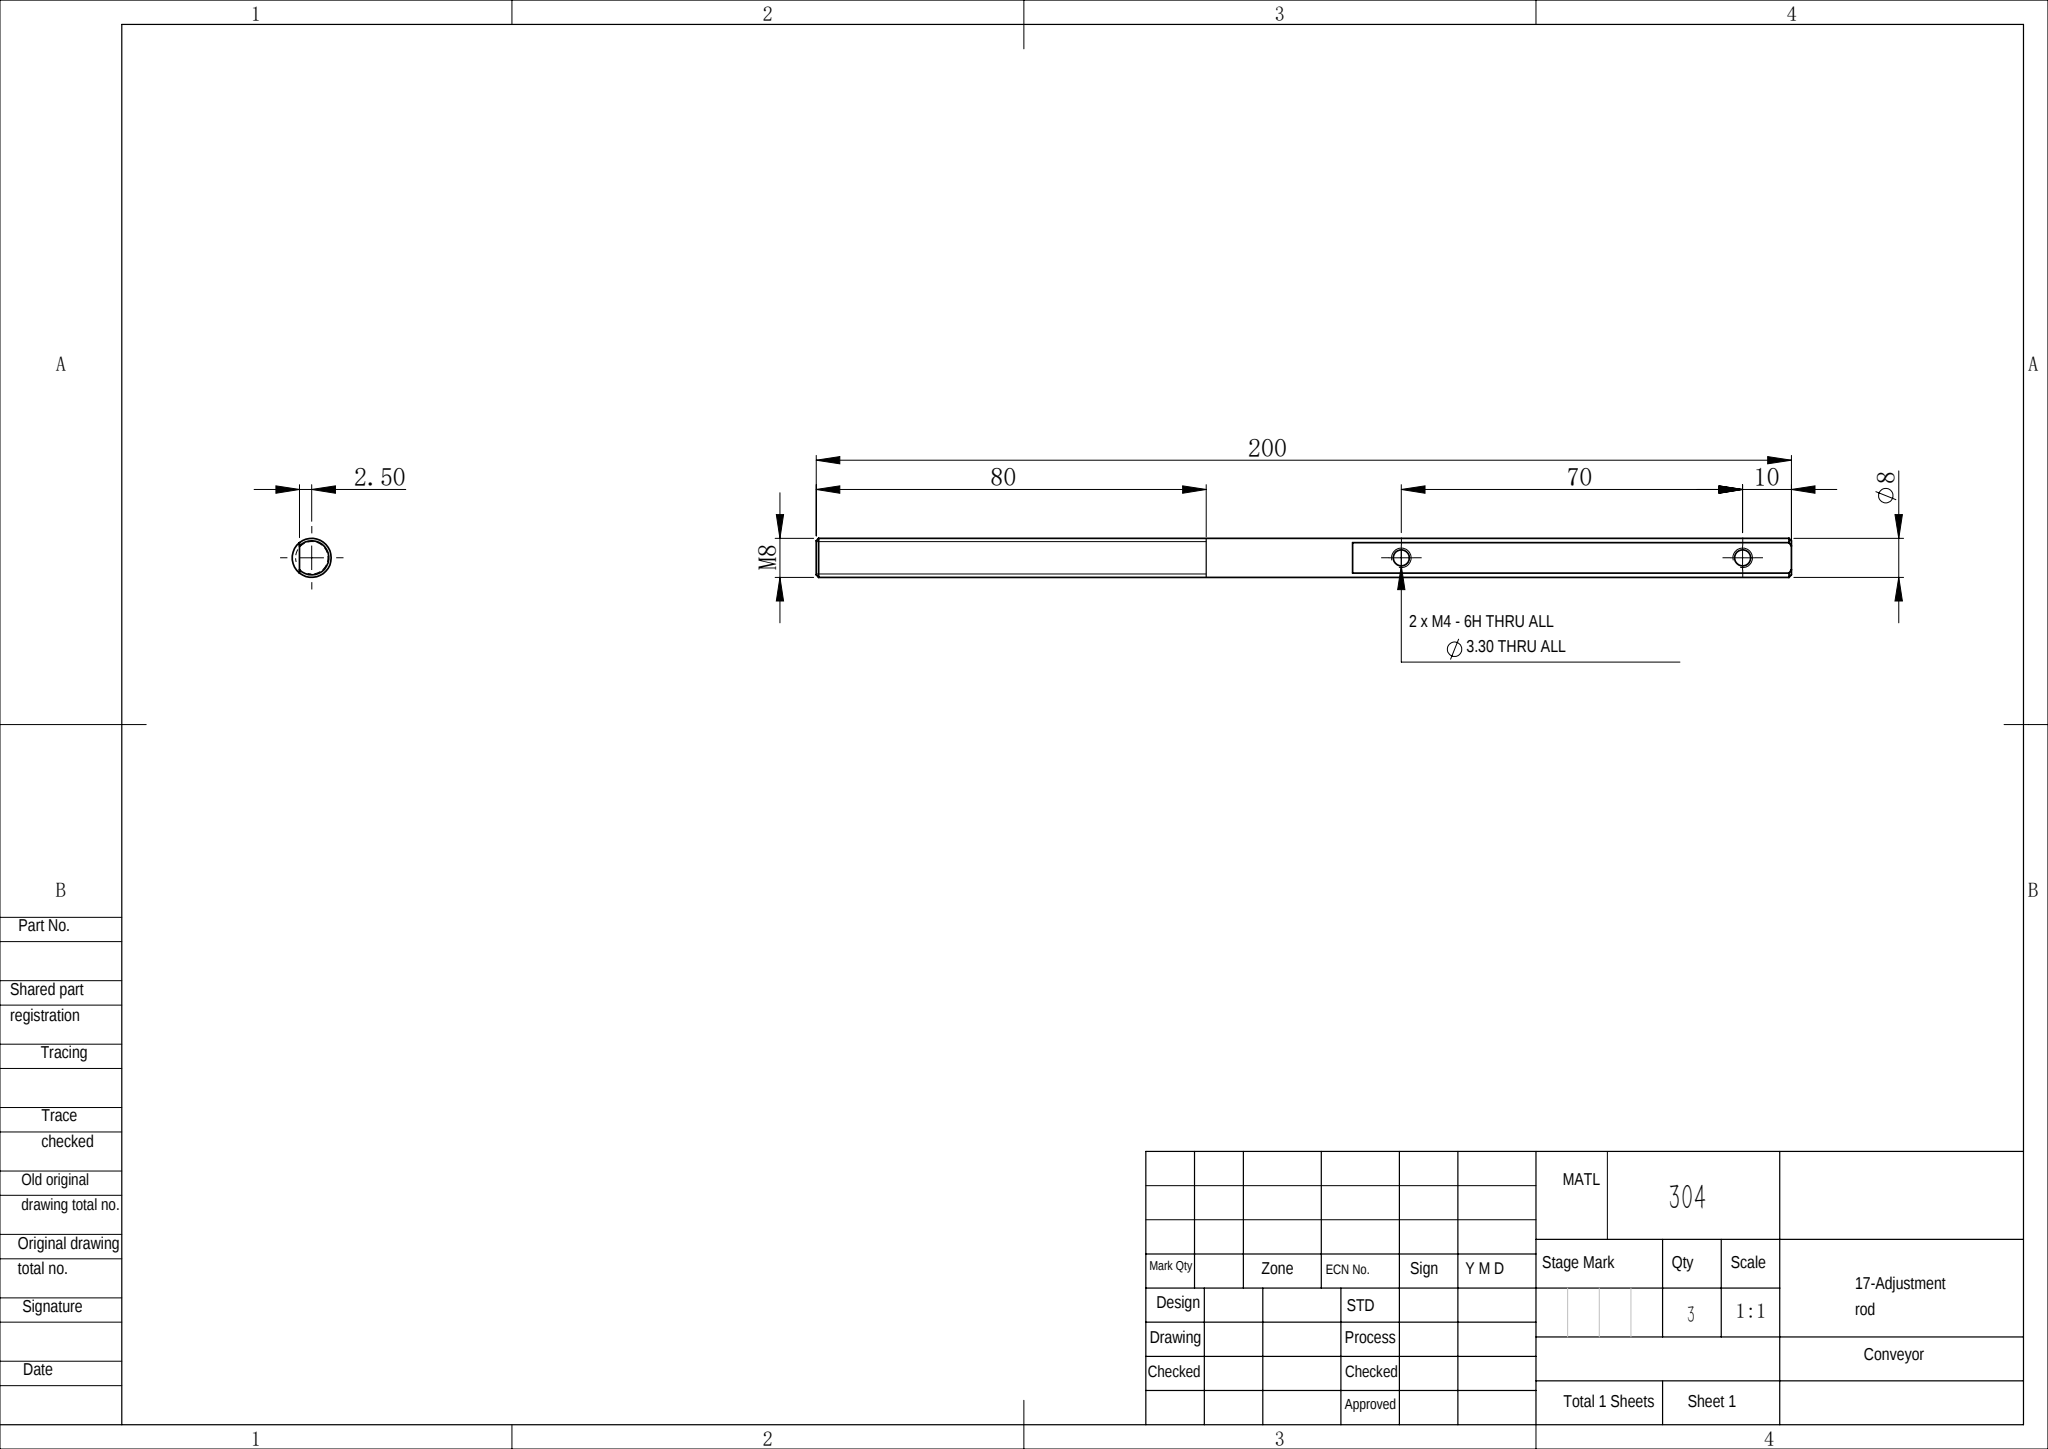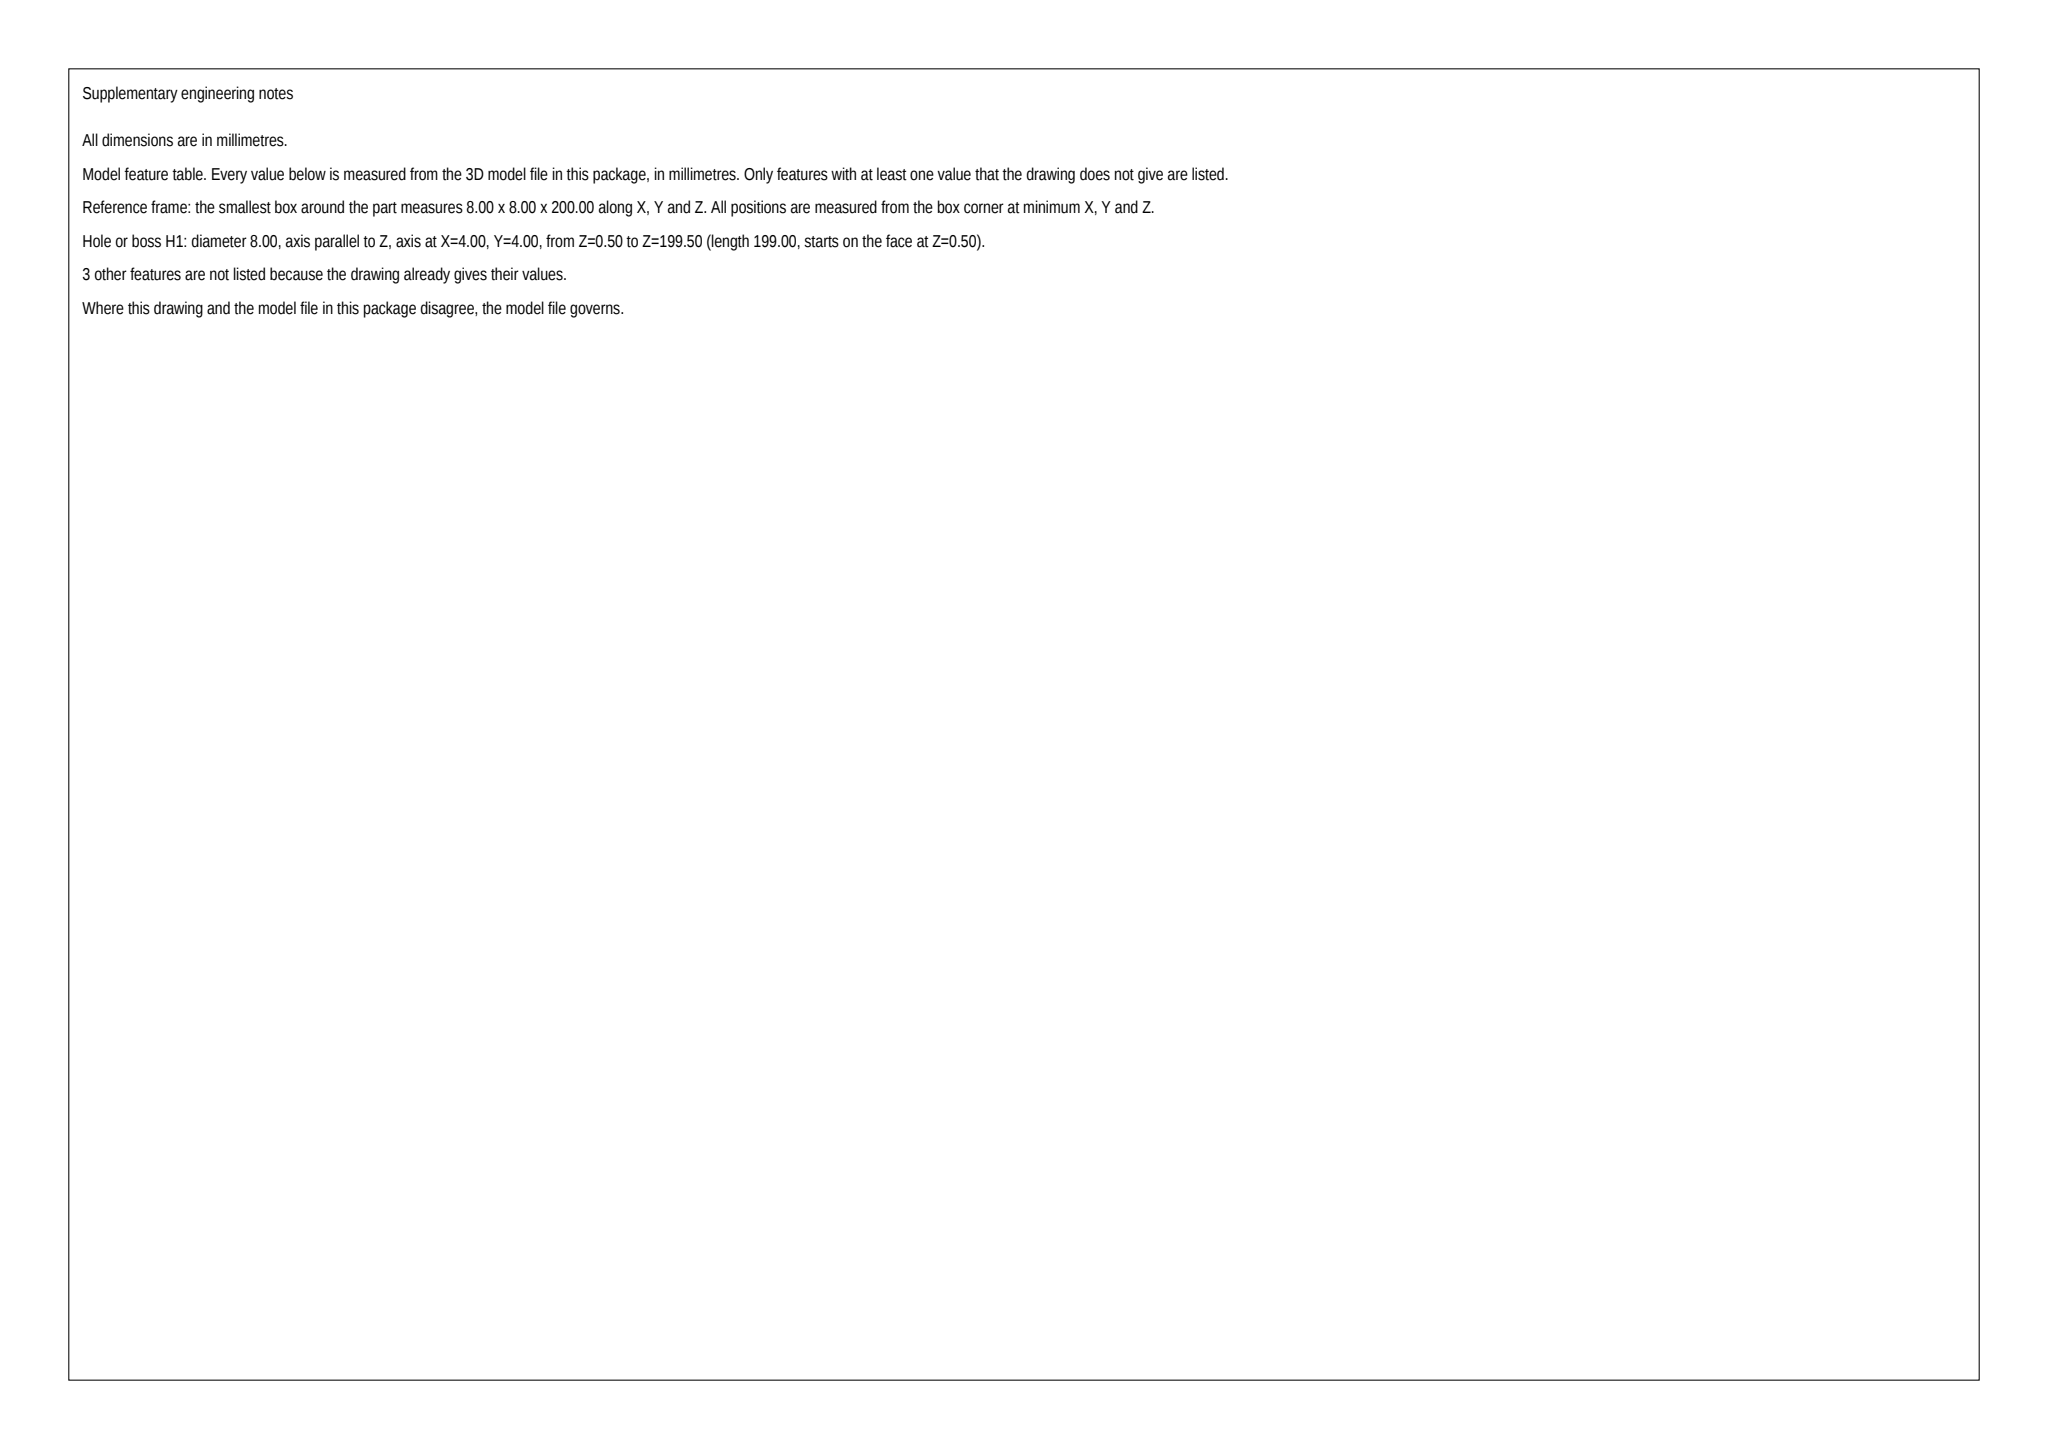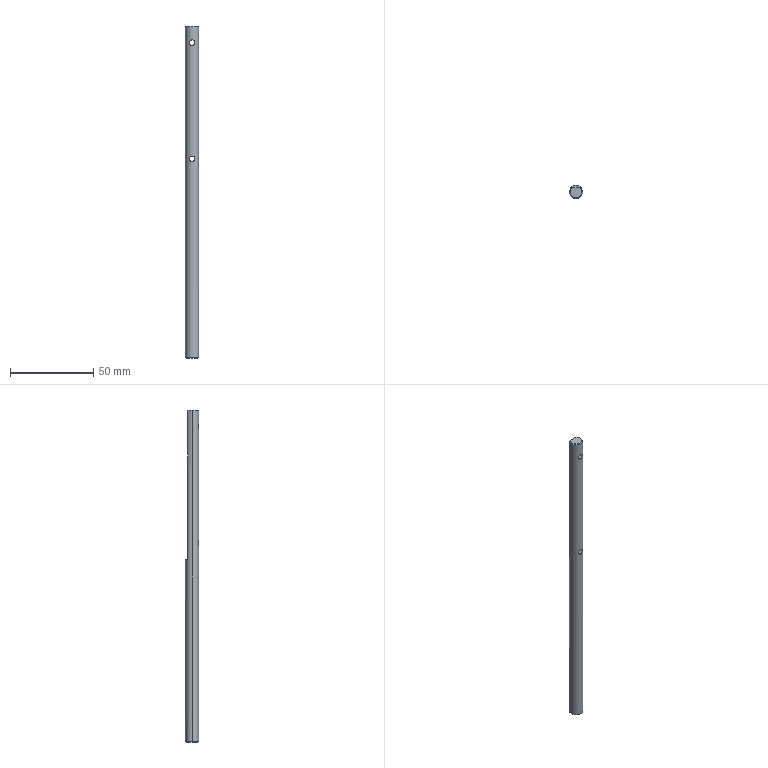Part | SolidWorks | mm | material 304 | 1 solid | 15 faces | box 8 x 8 x 200 mm | volume 9351 mm3 | cylinder 6 | cone 5 | plane 4 | commonest cylinder face diameters 3.3 x4 8 x2
build123d program:
from build123d import *

# Parameters (mm, degrees)
SKETCH1_R           = 4
BOSS_EXTRUDE1_DEPTH = 200
CHAMFER1_SIZE       = 0.5
SKETCH2_W           = 23.584
SKETCH2_H           = 6.641
CUT_EXTRUDE1_DEPTH  = 90
M4_TAPPED_HOLE1_D   = 3.3


with BuildPart() as part:
    # Sketch1 → Boss-Extrude1 (new body)
    with BuildSketch(Plane.XY):
        Circle(SKETCH1_R)
    extrude(amount=BOSS_EXTRUDE1_DEPTH)

    # Chamfer1
    chamfer1_edges = [part.edges().sort_by_distance(p)[0] for p in [
        (-4, 0, 0),
        (-4, 0, 200),
    ]]
    chamfer(chamfer1_edges, length=CHAMFER1_SIZE)

    # Sketch2 → Cut-Extrude1 (cut)
    with BuildSketch(Plane.XY.offset(200)):
        with Locations((0, 5.821)):
            Rectangle(SKETCH2_W, SKETCH2_H)
    extrude(amount=-CUT_EXTRUDE1_DEPTH, mode=Mode.SUBTRACT)

    # M4 Tapped Hole1 (through all)
    with Locations(Plane(origin=(0, 2.5, 0), x_dir=(1, 0, 0), z_dir=(0, 1, 0))):
        with Locations((0, -190), (0, -120)):
            Hole(M4_TAPPED_HOLE1_D / 2)


solid = part.part
STEP:
#1=CARTESIAN_POINT('',(-0.,-4.,118.35));
#2=VERTEX_POINT('',#1);
#3=CARTESIAN_POINT('',(-0.,-4.,121.65));
#4=VERTEX_POINT('',#3);
#5=CARTESIAN_POINT('',(-0.,-4.,118.35));
#6=CARTESIAN_POINT('',(-0.1086,-4.,118.35));
#7=CARTESIAN_POINT('',(-0.2188,-3.995,118.361));
#8=CARTESIAN_POINT('',(-0.4326,-3.978,118.404));
#9=CARTESIAN_POINT('',(-0.5359,-3.965,118.436));
#10=CARTESIAN_POINT('',(-0.8355,-3.917,118.561));
#11=CARTESIAN_POINT('',(-1.016,-3.872,118.682));
#12=CARTESIAN_POINT('',(-1.244,-3.803,118.91));
#13=CARTESIAN_POINT('',(-1.311,-3.78,118.992));
#14=CARTESIAN_POINT('',(-1.43,-3.736,119.17));
#15=CARTESIAN_POINT('',(-1.481,-3.716,119.266));
#16=CARTESIAN_POINT('',(-1.564,-3.682,119.465));
#17=CARTESIAN_POINT('',(-1.596,-3.668,119.567));
#18=CARTESIAN_POINT('',(-1.639,-3.649,119.78));
#19=CARTESIAN_POINT('',(-1.65,-3.644,119.891));
#20=CARTESIAN_POINT('',(-1.65,-3.644,120.217));
#21=CARTESIAN_POINT('',(-1.606,-3.665,120.436));
#22=CARTESIAN_POINT('',(-1.482,-3.716,120.734));
#23=CARTESIAN_POINT('',(-1.43,-3.736,120.83));
#24=CARTESIAN_POINT('',(-1.311,-3.78,121.008));
#25=CARTESIAN_POINT('',(-1.243,-3.803,121.09));
#26=CARTESIAN_POINT('',(-1.092,-3.849,121.242));
#27=CARTESIAN_POINT('',(-1.008,-3.872,121.311));
#28=CARTESIAN_POINT('',(-0.8311,-3.914,121.429));
#29=CARTESIAN_POINT('',(-0.7368,-3.933,121.48));
#30=CARTESIAN_POINT('',(-0.4348,-3.982,121.607));
#31=CARTESIAN_POINT('',(-0.2205,-4.,121.65));
#32=CARTESIAN_POINT('',(-0.,-4.,121.65));
#33=B_SPLINE_CURVE_WITH_KNOTS('',3,(#5,#6,#7,#8,#9,#10,#11,#12,#13,#14,#15,#16,#17,#18,#19,#20,#21,#22,#23,#24,#25,#26,#27,#28,#29,#30,#31,#32),.UNSPECIFIED.,.F.,.F.,(4,2,2,2,2,2,2,2,2,2,2,2,2,4),(0.005218,0.005543,0.005869,0.006521,0.006847,0.007173,0.007499,0.007824,0.008476,0.008802,0.009128,0.009454,0.009779,0.01043),.UNSPECIFIED.);
#34=EDGE_CURVE('',#2,#4,#33,.T.);
#35=ORIENTED_EDGE('',*,*,#34,.F.);
#36=CARTESIAN_POINT('',(-0.,2.5,118.35));
#37=VERTEX_POINT('',#36);
#38=CARTESIAN_POINT('',(-0.,2.5,118.35));
#39=DIRECTION('',(0.,1.,0.));
#40=VECTOR('',#39,1000.);
#41=LINE('',#38,#40);
#42=EDGE_CURVE('',#2,#37,#41,.T.);
#43=ORIENTED_EDGE('',*,*,#42,.T.);
#44=CARTESIAN_POINT('',(-0.,2.5,121.65));
#45=VERTEX_POINT('',#44);
#46=CARTESIAN_POINT('',(-0.,2.5,120.));
#47=DIRECTION('',(0.,1.,0.));
#48=DIRECTION('',(0.,0.,1.));
#49=AXIS2_PLACEMENT_3D('',#46,#47,#48);
#50=CIRCLE('',#49,1.65);
#51=EDGE_CURVE('',#37,#45,#50,.T.);
#52=ORIENTED_EDGE('',*,*,#51,.T.);
#53=CARTESIAN_POINT('',(-0.,2.5,121.65));
#54=DIRECTION('',(0.,1.,0.));
#55=VECTOR('',#54,1000.);
#56=LINE('',#53,#55);
#57=EDGE_CURVE('',#4,#45,#56,.T.);
#58=ORIENTED_EDGE('',*,*,#57,.F.);
#59=EDGE_LOOP('',(#35,#43,#52,#58));
#60=FACE_OUTER_BOUND('',#59,.T.);
#61=CARTESIAN_POINT('',(-0.,2.5,120.));
#62=DIRECTION('',(0.,1.,0.));
#63=DIRECTION('',(0.,0.,1.));
#64=AXIS2_PLACEMENT_3D('',#61,#62,#63);
#65=CYLINDRICAL_SURFACE('',#64,1.65);
#66=ADVANCED_FACE('',(#60),#65,.F.);
#67=CARTESIAN_POINT('',(0.,-4.,188.35));
#68=VERTEX_POINT('',#67);
#69=CARTESIAN_POINT('',(0.,-4.,191.65));
#70=VERTEX_POINT('',#69);
#71=CARTESIAN_POINT('',(0.,-4.,188.35));
#72=CARTESIAN_POINT('',(-0.1086,-4.,188.35));
#73=CARTESIAN_POINT('',(-0.2188,-3.995,188.361));
#74=CARTESIAN_POINT('',(-0.4326,-3.978,188.404));
#75=CARTESIAN_POINT('',(-0.5359,-3.965,188.436));
#76=CARTESIAN_POINT('',(-0.8355,-3.917,188.561));
#77=CARTESIAN_POINT('',(-1.016,-3.872,188.682));
#78=CARTESIAN_POINT('',(-1.244,-3.803,188.91));
#79=CARTESIAN_POINT('',(-1.311,-3.78,188.992));
#80=CARTESIAN_POINT('',(-1.43,-3.736,189.17));
#81=CARTESIAN_POINT('',(-1.481,-3.716,189.266));
#82=CARTESIAN_POINT('',(-1.564,-3.682,189.465));
#83=CARTESIAN_POINT('',(-1.596,-3.668,189.567));
#84=CARTESIAN_POINT('',(-1.639,-3.649,189.78));
#85=CARTESIAN_POINT('',(-1.65,-3.644,189.891));
#86=CARTESIAN_POINT('',(-1.65,-3.644,190.217));
#87=CARTESIAN_POINT('',(-1.606,-3.665,190.436));
#88=CARTESIAN_POINT('',(-1.482,-3.716,190.734));
#89=CARTESIAN_POINT('',(-1.43,-3.736,190.83));
#90=CARTESIAN_POINT('',(-1.311,-3.78,191.008));
#91=CARTESIAN_POINT('',(-1.243,-3.803,191.09));
#92=CARTESIAN_POINT('',(-1.092,-3.849,191.242));
#93=CARTESIAN_POINT('',(-1.008,-3.872,191.311));
#94=CARTESIAN_POINT('',(-0.8311,-3.914,191.429));
#95=CARTESIAN_POINT('',(-0.7368,-3.933,191.48));
#96=CARTESIAN_POINT('',(-0.4348,-3.982,191.607));
#97=CARTESIAN_POINT('',(-0.2205,-4.,191.65));
#98=CARTESIAN_POINT('',(0.,-4.,191.65));
#99=B_SPLINE_CURVE_WITH_KNOTS('',3,(#71,#72,#73,#74,#75,#76,#77,#78,#79,#80,#81,#82,#83,#84,#85,#86,#87,#88,#89,#90,#91,#92,#93,#94,#95,#96,#97,#98),.UNSPECIFIED.,.F.,.F.,(4,2,2,2,2,2,2,2,2,2,2,2,2,4),(0.005218,0.005543,0.005869,0.006521,0.006847,0.007173,0.007499,0.007824,0.008476,0.008802,0.009128,0.009454,0.009779,0.01043),.UNSPECIFIED.);
#100=EDGE_CURVE('',#68,#70,#99,.T.);
#101=ORIENTED_EDGE('',*,*,#100,.F.);
#102=CARTESIAN_POINT('',(0.,2.5,188.35));
#103=VERTEX_POINT('',#102);
#104=CARTESIAN_POINT('',(0.,2.5,188.35));
#105=DIRECTION('',(0.,1.,0.));
#106=VECTOR('',#105,1000.);
#107=LINE('',#104,#106);
#108=EDGE_CURVE('',#68,#103,#107,.T.);
#109=ORIENTED_EDGE('',*,*,#108,.T.);
#110=CARTESIAN_POINT('',(0.,2.5,191.65));
#111=VERTEX_POINT('',#110);
#112=CARTESIAN_POINT('',(0.,2.5,190.));
#113=DIRECTION('',(0.,1.,0.));
#114=DIRECTION('',(0.,0.,1.));
#115=AXIS2_PLACEMENT_3D('',#112,#113,#114);
#116=CIRCLE('',#115,1.65);
#117=EDGE_CURVE('',#103,#111,#116,.T.);
#118=ORIENTED_EDGE('',*,*,#117,.T.);
#119=CARTESIAN_POINT('',(0.,2.5,191.65));
#120=DIRECTION('',(0.,1.,0.));
#121=VECTOR('',#120,1000.);
#122=LINE('',#119,#121);
#123=EDGE_CURVE('',#70,#111,#122,.T.);
#124=ORIENTED_EDGE('',*,*,#123,.F.);
#125=EDGE_LOOP('',(#101,#109,#118,#124));
#126=FACE_OUTER_BOUND('',#125,.T.);
#127=CARTESIAN_POINT('',(0.,2.5,190.));
#128=DIRECTION('',(0.,1.,0.));
#129=DIRECTION('',(0.,0.,1.));
#130=AXIS2_PLACEMENT_3D('',#127,#128,#129);
#131=CYLINDRICAL_SURFACE('',#130,1.65);
#132=ADVANCED_FACE('',(#126),#131,.F.);
#133=CARTESIAN_POINT('',(-3.5,0.,0.));
#134=VERTEX_POINT('',#133);
#135=CARTESIAN_POINT('',(3.5,0.,0.));
#136=VERTEX_POINT('',#135);
#137=CARTESIAN_POINT('',(0.,0.,0.));
#138=DIRECTION('',(0.,0.,-1.));
#139=DIRECTION('',(1.,0.,0.));
#140=AXIS2_PLACEMENT_3D('',#137,#138,#139);
#141=CIRCLE('',#140,3.5);
#142=EDGE_CURVE('',#134,#136,#141,.T.);
#143=ORIENTED_EDGE('',*,*,#142,.F.);
#144=CARTESIAN_POINT('',(-4.,0.,0.5));
#145=VERTEX_POINT('',#144);
#146=CARTESIAN_POINT('',(-4.,0.,0.5));
#147=DIRECTION('',(-0.7071,0.,0.7071));
#148=VECTOR('',#147,1000.);
#149=LINE('',#146,#148);
#150=EDGE_CURVE('',#134,#145,#149,.T.);
#151=ORIENTED_EDGE('',*,*,#150,.T.);
#152=CARTESIAN_POINT('',(4.,0.,0.5));
#153=VERTEX_POINT('',#152);
#154=CARTESIAN_POINT('',(0.,0.,0.5));
#155=DIRECTION('',(0.,0.,1.));
#156=DIRECTION('',(1.,0.,0.));
#157=AXIS2_PLACEMENT_3D('',#154,#155,#156);
#158=CIRCLE('',#157,4.);
#159=EDGE_CURVE('',#153,#145,#158,.T.);
#160=ORIENTED_EDGE('',*,*,#159,.F.);
#161=CARTESIAN_POINT('',(4.,0.,0.5));
#162=DIRECTION('',(0.7071,0.,0.7071));
#163=VECTOR('',#162,1000.);
#164=LINE('',#161,#163);
#165=EDGE_CURVE('',#136,#153,#164,.T.);
#166=ORIENTED_EDGE('',*,*,#165,.F.);
#167=EDGE_LOOP('',(#143,#151,#160,#166));
#168=FACE_OUTER_BOUND('',#167,.T.);
#169=CARTESIAN_POINT('',(0.,0.,0.5));
#170=DIRECTION('',(0.,0.,1.));
#171=DIRECTION('',(1.,0.,0.));
#172=AXIS2_PLACEMENT_3D('',#169,#170,#171);
#173=CONICAL_SURFACE('',#172,4.,0.7854);
#174=ADVANCED_FACE('',(#168),#173,.T.);
#175=CARTESIAN_POINT('',(3.5,0.,200.));
#176=VERTEX_POINT('',#175);
#177=CARTESIAN_POINT('',(2.449,2.5,200.));
#178=VERTEX_POINT('',#177);
#179=CARTESIAN_POINT('',(0.,0.,200.));
#180=DIRECTION('',(0.,0.,1.));
#181=DIRECTION('',(1.,0.,0.));
#182=AXIS2_PLACEMENT_3D('',#179,#180,#181);
#183=CIRCLE('',#182,3.5);
#184=EDGE_CURVE('',#176,#178,#183,.T.);
#185=ORIENTED_EDGE('',*,*,#184,.F.);
#186=CARTESIAN_POINT('',(4.,0.,199.5));
#187=VERTEX_POINT('',#186);
#188=CARTESIAN_POINT('',(3.5,0.,200.));
#189=DIRECTION('',(0.7071,0.,-0.7071));
#190=VECTOR('',#189,1000.);
#191=LINE('',#188,#190);
#192=EDGE_CURVE('',#176,#187,#191,.T.);
#193=ORIENTED_EDGE('',*,*,#192,.T.);
#194=CARTESIAN_POINT('',(3.122,2.5,199.5));
#195=VERTEX_POINT('',#194);
#196=CARTESIAN_POINT('',(0.,0.,199.5));
#197=DIRECTION('',(0.,0.,-1.));
#198=DIRECTION('',(1.,0.,0.));
#199=AXIS2_PLACEMENT_3D('',#196,#197,#198);
#200=CIRCLE('',#199,4.);
#201=EDGE_CURVE('',#195,#187,#200,.T.);
#202=ORIENTED_EDGE('',*,*,#201,.F.);
#203=CARTESIAN_POINT('',(2.449,2.5,200.));
#204=CARTESIAN_POINT('',(2.678,2.5,199.84));
#205=CARTESIAN_POINT('',(2.902,2.5,199.672));
#206=CARTESIAN_POINT('',(3.122,2.5,199.5));
#207=B_SPLINE_CURVE_WITH_KNOTS('',3,(#203,#204,#205,#206),.UNSPECIFIED.,.F.,.F.,(4,4),(0.0134,0.01424),.UNSPECIFIED.);
#208=EDGE_CURVE('',#178,#195,#207,.T.);
#209=ORIENTED_EDGE('',*,*,#208,.F.);
#210=EDGE_LOOP('',(#185,#193,#202,#209));
#211=FACE_OUTER_BOUND('',#210,.T.);
#212=CARTESIAN_POINT('',(0.,0.,200.));
#213=DIRECTION('',(0.,0.,-1.));
#214=DIRECTION('',(-1.,0.,0.));
#215=AXIS2_PLACEMENT_3D('',#212,#213,#214);
#216=CONICAL_SURFACE('',#215,3.5,0.7854);
#217=ADVANCED_FACE('',(#211),#216,.T.);
#218=ORIENTED_EDGE('',*,*,#192,.F.);
#219=CARTESIAN_POINT('',(-3.5,0.,200.));
#220=VERTEX_POINT('',#219);
#221=CARTESIAN_POINT('',(0.,0.,200.));
#222=DIRECTION('',(0.,0.,1.));
#223=DIRECTION('',(1.,0.,0.));
#224=AXIS2_PLACEMENT_3D('',#221,#222,#223);
#225=CIRCLE('',#224,3.5);
#226=EDGE_CURVE('',#220,#176,#225,.T.);
#227=ORIENTED_EDGE('',*,*,#226,.F.);
#228=CARTESIAN_POINT('',(-4.,0.,199.5));
#229=VERTEX_POINT('',#228);
#230=CARTESIAN_POINT('',(-3.5,0.,200.));
#231=DIRECTION('',(-0.7071,0.,-0.7071));
#232=VECTOR('',#231,1000.);
#233=LINE('',#230,#232);
#234=EDGE_CURVE('',#220,#229,#233,.T.);
#235=ORIENTED_EDGE('',*,*,#234,.T.);
#236=CARTESIAN_POINT('',(0.,0.,199.5));
#237=DIRECTION('',(0.,0.,-1.));
#238=DIRECTION('',(1.,0.,0.));
#239=AXIS2_PLACEMENT_3D('',#236,#237,#238);
#240=CIRCLE('',#239,4.);
#241=EDGE_CURVE('',#187,#229,#240,.T.);
#242=ORIENTED_EDGE('',*,*,#241,.F.);
#243=EDGE_LOOP('',(#218,#227,#235,#242));
#244=FACE_OUTER_BOUND('',#243,.T.);
#245=CARTESIAN_POINT('',(0.,0.,200.));
#246=DIRECTION('',(0.,0.,-1.));
#247=DIRECTION('',(-1.,0.,0.));
#248=AXIS2_PLACEMENT_3D('',#245,#246,#247);
#249=CONICAL_SURFACE('',#248,3.5,0.7854);
#250=ADVANCED_FACE('',(#244),#249,.T.);
#251=ORIENTED_EDGE('',*,*,#201,.T.);
#252=CARTESIAN_POINT('',(4.,0.,200.));
#253=DIRECTION('',(0.,0.,-1.));
#254=VECTOR('',#253,1000.);
#255=LINE('',#252,#254);
#256=EDGE_CURVE('',#187,#153,#255,.T.);
#257=ORIENTED_EDGE('',*,*,#256,.T.);
#258=ORIENTED_EDGE('',*,*,#159,.T.);
#259=CARTESIAN_POINT('',(-4.,0.,200.));
#260=DIRECTION('',(0.,0.,-1.));
#261=VECTOR('',#260,1000.);
#262=LINE('',#259,#261);
#263=EDGE_CURVE('',#229,#145,#262,.T.);
#264=ORIENTED_EDGE('',*,*,#263,.F.);
#265=CARTESIAN_POINT('',(-3.122,2.5,199.5));
#266=VERTEX_POINT('',#265);
#267=CARTESIAN_POINT('',(0.,0.,199.5));
#268=DIRECTION('',(0.,0.,-1.));
#269=DIRECTION('',(1.,0.,0.));
#270=AXIS2_PLACEMENT_3D('',#267,#268,#269);
#271=CIRCLE('',#270,4.);
#272=EDGE_CURVE('',#229,#266,#271,.T.);
#273=ORIENTED_EDGE('',*,*,#272,.T.);
#274=CARTESIAN_POINT('',(-3.122,2.5,110.));
#275=VERTEX_POINT('',#274);
#276=CARTESIAN_POINT('',(-3.122,2.5,200.));
#277=DIRECTION('',(0.,0.,-1.));
#278=VECTOR('',#277,1000.);
#279=LINE('',#276,#278);
#280=EDGE_CURVE('',#266,#275,#279,.T.);
#281=ORIENTED_EDGE('',*,*,#280,.T.);
#282=CARTESIAN_POINT('',(3.122,2.5,110.));
#283=VERTEX_POINT('',#282);
#284=CARTESIAN_POINT('',(0.,0.,110.));
#285=DIRECTION('',(0.,0.,1.));
#286=DIRECTION('',(1.,0.,0.));
#287=AXIS2_PLACEMENT_3D('',#284,#285,#286);
#288=CIRCLE('',#287,4.);
#289=EDGE_CURVE('',#283,#275,#288,.T.);
#290=ORIENTED_EDGE('',*,*,#289,.F.);
#291=CARTESIAN_POINT('',(3.122,2.5,200.));
#292=DIRECTION('',(0.,0.,1.));
#293=VECTOR('',#292,1000.);
#294=LINE('',#291,#293);
#295=EDGE_CURVE('',#283,#195,#294,.T.);
#296=ORIENTED_EDGE('',*,*,#295,.T.);
#297=EDGE_LOOP('',(#251,#257,#258,#264,#273,#281,#290,#296));
#298=FACE_OUTER_BOUND('',#297,.T.);
#299=CARTESIAN_POINT('',(0.,0.,200.));
#300=DIRECTION('',(0.,0.,-1.));
#301=DIRECTION('',(-1.,0.,0.));
#302=AXIS2_PLACEMENT_3D('',#299,#300,#301);
#303=CYLINDRICAL_SURFACE('',#302,4.);
#304=ADVANCED_FACE('',(#298),#303,.T.);
#305=ORIENTED_EDGE('',*,*,#256,.F.);
#306=ORIENTED_EDGE('',*,*,#241,.T.);
#307=ORIENTED_EDGE('',*,*,#263,.T.);
#308=CARTESIAN_POINT('',(0.,0.,0.5));
#309=DIRECTION('',(0.,0.,1.));
#310=DIRECTION('',(1.,0.,0.));
#311=AXIS2_PLACEMENT_3D('',#308,#309,#310);
#312=CIRCLE('',#311,4.);
#313=EDGE_CURVE('',#145,#153,#312,.T.);
#314=ORIENTED_EDGE('',*,*,#313,.T.);
#315=EDGE_LOOP('',(#305,#306,#307,#314));
#316=FACE_OUTER_BOUND('',#315,.T.);
#317=CARTESIAN_POINT('',(-0.,-4.,121.65));
#318=CARTESIAN_POINT('',(0.1103,-4.,121.65));
#319=CARTESIAN_POINT('',(0.2186,-3.995,121.639));
#320=CARTESIAN_POINT('',(0.4313,-3.978,121.596));
#321=CARTESIAN_POINT('',(0.5367,-3.965,121.564));
#322=CARTESIAN_POINT('',(0.8358,-3.917,121.439));
#323=CARTESIAN_POINT('',(1.017,-3.872,121.316));
#324=CARTESIAN_POINT('',(1.318,-3.78,121.015));
#325=CARTESIAN_POINT('',(1.44,-3.733,120.834));
#326=CARTESIAN_POINT('',(1.564,-3.682,120.537));
#327=CARTESIAN_POINT('',(1.596,-3.668,120.432));
#328=CARTESIAN_POINT('',(1.639,-3.649,120.218));
#329=CARTESIAN_POINT('',(1.65,-3.644,120.11));
#330=CARTESIAN_POINT('',(1.65,-3.644,119.892));
#331=CARTESIAN_POINT('',(1.639,-3.649,119.781));
#332=CARTESIAN_POINT('',(1.596,-3.668,119.569));
#333=CARTESIAN_POINT('',(1.565,-3.682,119.465));
#334=CARTESIAN_POINT('',(1.481,-3.716,119.264));
#335=CARTESIAN_POINT('',(1.43,-3.736,119.17));
#336=CARTESIAN_POINT('',(1.311,-3.78,118.992));
#337=CARTESIAN_POINT('',(1.242,-3.803,118.908));
#338=CARTESIAN_POINT('',(1.091,-3.849,118.757));
#339=CARTESIAN_POINT('',(1.009,-3.872,118.69));
#340=CARTESIAN_POINT('',(0.8304,-3.914,118.57));
#341=CARTESIAN_POINT('',(0.7343,-3.933,118.519));
#342=CARTESIAN_POINT('',(0.4369,-3.981,118.394));
#343=CARTESIAN_POINT('',(0.2174,-4.,118.35));
#344=CARTESIAN_POINT('',(-0.,-4.,118.35));
#345=B_SPLINE_CURVE_WITH_KNOTS('',3,(#317,#318,#319,#320,#321,#322,#323,#324,#325,#326,#327,#328,#329,#330,#331,#332,#333,#334,#335,#336,#337,#338,#339,#340,#341,#342,#343,#344),.UNSPECIFIED.,.F.,.F.,(4,2,2,2,2,2,2,2,2,2,2,2,2,4),(0.,0.0003261,0.0006522,0.001304,0.001957,0.002283,0.002609,0.002935,0.003261,0.003587,0.003913,0.004239,0.004565,0.005218),.UNSPECIFIED.);
#346=EDGE_CURVE('',#4,#2,#345,.T.);
#347=ORIENTED_EDGE('',*,*,#346,.T.);
#348=ORIENTED_EDGE('',*,*,#34,.T.);
#349=EDGE_LOOP('',(#347,#348));
#350=FACE_BOUND('',#349,.T.);
#351=CARTESIAN_POINT('',(0.,-4.,191.65));
#352=CARTESIAN_POINT('',(0.1103,-4.,191.65));
#353=CARTESIAN_POINT('',(0.2186,-3.995,191.639));
#354=CARTESIAN_POINT('',(0.4313,-3.978,191.596));
#355=CARTESIAN_POINT('',(0.5367,-3.965,191.564));
#356=CARTESIAN_POINT('',(0.8358,-3.917,191.439));
#357=CARTESIAN_POINT('',(1.017,-3.872,191.316));
#358=CARTESIAN_POINT('',(1.318,-3.78,191.015));
#359=CARTESIAN_POINT('',(1.44,-3.733,190.834));
#360=CARTESIAN_POINT('',(1.564,-3.682,190.537));
#361=CARTESIAN_POINT('',(1.596,-3.668,190.432));
#362=CARTESIAN_POINT('',(1.639,-3.649,190.218));
#363=CARTESIAN_POINT('',(1.65,-3.644,190.11));
#364=CARTESIAN_POINT('',(1.65,-3.644,189.892));
#365=CARTESIAN_POINT('',(1.639,-3.649,189.781));
#366=CARTESIAN_POINT('',(1.596,-3.668,189.569));
#367=CARTESIAN_POINT('',(1.565,-3.682,189.465));
#368=CARTESIAN_POINT('',(1.481,-3.716,189.264));
#369=CARTESIAN_POINT('',(1.43,-3.736,189.17));
#370=CARTESIAN_POINT('',(1.311,-3.78,188.992));
#371=CARTESIAN_POINT('',(1.242,-3.803,188.908));
#372=CARTESIAN_POINT('',(1.091,-3.849,188.757));
#373=CARTESIAN_POINT('',(1.009,-3.872,188.69));
#374=CARTESIAN_POINT('',(0.8304,-3.914,188.57));
#375=CARTESIAN_POINT('',(0.7343,-3.933,188.519));
#376=CARTESIAN_POINT('',(0.4369,-3.981,188.394));
#377=CARTESIAN_POINT('',(0.2174,-4.,188.35));
#378=CARTESIAN_POINT('',(0.,-4.,188.35));
#379=B_SPLINE_CURVE_WITH_KNOTS('',3,(#351,#352,#353,#354,#355,#356,#357,#358,#359,#360,#361,#362,#363,#364,#365,#366,#367,#368,#369,#370,#371,#372,#373,#374,#375,#376,#377,#378),.UNSPECIFIED.,.F.,.F.,(4,2,2,2,2,2,2,2,2,2,2,2,2,4),(0.,0.0003261,0.0006522,0.001304,0.001957,0.002283,0.002609,0.002935,0.003261,0.003587,0.003913,0.004239,0.004565,0.005218),.UNSPECIFIED.);
#380=EDGE_CURVE('',#70,#68,#379,.T.);
#381=ORIENTED_EDGE('',*,*,#380,.T.);
#382=ORIENTED_EDGE('',*,*,#100,.T.);
#383=EDGE_LOOP('',(#381,#382));
#384=FACE_BOUND('',#383,.T.);
#385=CARTESIAN_POINT('',(0.,0.,200.));
#386=DIRECTION('',(0.,0.,-1.));
#387=DIRECTION('',(-1.,0.,0.));
#388=AXIS2_PLACEMENT_3D('',#385,#386,#387);
#389=CYLINDRICAL_SURFACE('',#388,4.);
#390=ADVANCED_FACE('',(#316,#350,#384),#389,.T.);
#391=CARTESIAN_POINT('',(-2.449,2.5,200.));
#392=VERTEX_POINT('',#391);
#393=CARTESIAN_POINT('',(11.792,2.5,200.));
#394=DIRECTION('',(1.,0.,0.));
#395=VECTOR('',#394,1000.);
#396=LINE('',#393,#395);
#397=EDGE_CURVE('',#392,#178,#396,.T.);
#398=ORIENTED_EDGE('',*,*,#397,.F.);
#399=CARTESIAN_POINT('',(0.,0.,200.));
#400=DIRECTION('',(0.,0.,1.));
#401=DIRECTION('',(1.,0.,0.));
#402=AXIS2_PLACEMENT_3D('',#399,#400,#401);
#403=CIRCLE('',#402,3.5);
#404=EDGE_CURVE('',#392,#220,#403,.T.);
#405=ORIENTED_EDGE('',*,*,#404,.T.);
#406=ORIENTED_EDGE('',*,*,#226,.T.);
#407=ORIENTED_EDGE('',*,*,#184,.T.);
#408=EDGE_LOOP('',(#398,#405,#406,#407));
#409=FACE_OUTER_BOUND('',#408,.T.);
#410=CARTESIAN_POINT('',(0.,0.,200.));
#411=DIRECTION('',(0.,0.,1.));
#412=DIRECTION('',(1.,0.,0.));
#413=AXIS2_PLACEMENT_3D('',#410,#411,#412);
#414=PLANE('',#413);
#415=ADVANCED_FACE('',(#409),#414,.T.);
#416=CARTESIAN_POINT('',(0.,0.,0.));
#417=DIRECTION('',(0.,0.,-1.));
#418=DIRECTION('',(1.,0.,0.));
#419=AXIS2_PLACEMENT_3D('',#416,#417,#418);
#420=CIRCLE('',#419,3.5);
#421=EDGE_CURVE('',#136,#134,#420,.T.);
#422=ORIENTED_EDGE('',*,*,#421,.T.);
#423=ORIENTED_EDGE('',*,*,#142,.T.);
#424=EDGE_LOOP('',(#422,#423));
#425=FACE_OUTER_BOUND('',#424,.T.);
#426=CARTESIAN_POINT('',(0.,0.,0.));
#427=DIRECTION('',(0.,0.,1.));
#428=DIRECTION('',(1.,0.,0.));
#429=AXIS2_PLACEMENT_3D('',#426,#427,#428);
#430=PLANE('',#429);
#431=ADVANCED_FACE('',(#425),#430,.F.);
#432=ORIENTED_EDGE('',*,*,#234,.F.);
#433=ORIENTED_EDGE('',*,*,#404,.F.);
#434=CARTESIAN_POINT('',(-3.122,2.5,199.5));
#435=CARTESIAN_POINT('',(-2.902,2.5,199.672));
#436=CARTESIAN_POINT('',(-2.678,2.5,199.84));
#437=CARTESIAN_POINT('',(-2.449,2.5,200.));
#438=B_SPLINE_CURVE_WITH_KNOTS('',3,(#434,#435,#436,#437),.UNSPECIFIED.,.F.,.F.,(4,4),(0.007178,0.008016),.UNSPECIFIED.);
#439=EDGE_CURVE('',#266,#392,#438,.T.);
#440=ORIENTED_EDGE('',*,*,#439,.F.);
#441=ORIENTED_EDGE('',*,*,#272,.F.);
#442=EDGE_LOOP('',(#432,#433,#440,#441));
#443=FACE_OUTER_BOUND('',#442,.T.);
#444=CARTESIAN_POINT('',(0.,0.,200.));
#445=DIRECTION('',(0.,0.,-1.));
#446=DIRECTION('',(-1.,0.,0.));
#447=AXIS2_PLACEMENT_3D('',#444,#445,#446);
#448=CONICAL_SURFACE('',#447,3.5,0.7854);
#449=ADVANCED_FACE('',(#443),#448,.T.);
#450=ORIENTED_EDGE('',*,*,#150,.F.);
#451=ORIENTED_EDGE('',*,*,#421,.F.);
#452=ORIENTED_EDGE('',*,*,#165,.T.);
#453=ORIENTED_EDGE('',*,*,#313,.F.);
#454=EDGE_LOOP('',(#450,#451,#452,#453));
#455=FACE_OUTER_BOUND('',#454,.T.);
#456=CARTESIAN_POINT('',(0.,0.,0.5));
#457=DIRECTION('',(0.,0.,1.));
#458=DIRECTION('',(1.,0.,0.));
#459=AXIS2_PLACEMENT_3D('',#456,#457,#458);
#460=CONICAL_SURFACE('',#459,4.,0.7854);
#461=ADVANCED_FACE('',(#455),#460,.T.);
#462=ORIENTED_EDGE('',*,*,#289,.T.);
#463=CARTESIAN_POINT('',(11.792,2.5,110.));
#464=DIRECTION('',(1.,0.,0.));
#465=VECTOR('',#464,1000.);
#466=LINE('',#463,#465);
#467=EDGE_CURVE('',#275,#283,#466,.T.);
#468=ORIENTED_EDGE('',*,*,#467,.T.);
#469=EDGE_LOOP('',(#462,#468));
#470=FACE_OUTER_BOUND('',#469,.T.);
#471=CARTESIAN_POINT('',(0.,0.,110.));
#472=DIRECTION('',(0.,0.,1.));
#473=DIRECTION('',(1.,0.,0.));
#474=AXIS2_PLACEMENT_3D('',#471,#472,#473);
#475=PLANE('',#474);
#476=ADVANCED_FACE('',(#470),#475,.T.);
#477=CARTESIAN_POINT('',(-0.,2.5,120.));
#478=DIRECTION('',(0.,1.,0.));
#479=DIRECTION('',(0.,0.,1.));
#480=AXIS2_PLACEMENT_3D('',#477,#478,#479);
#481=CIRCLE('',#480,1.65);
#482=EDGE_CURVE('',#45,#37,#481,.T.);
#483=ORIENTED_EDGE('',*,*,#482,.F.);
#484=ORIENTED_EDGE('',*,*,#51,.F.);
#485=EDGE_LOOP('',(#483,#484));
#486=FACE_BOUND('',#485,.T.);
#487=CARTESIAN_POINT('',(0.,2.5,190.));
#488=DIRECTION('',(0.,1.,0.));
#489=DIRECTION('',(0.,0.,1.));
#490=AXIS2_PLACEMENT_3D('',#487,#488,#489);
#491=CIRCLE('',#490,1.65);
#492=EDGE_CURVE('',#111,#103,#491,.T.);
#493=ORIENTED_EDGE('',*,*,#492,.F.);
#494=ORIENTED_EDGE('',*,*,#117,.F.);
#495=EDGE_LOOP('',(#493,#494));
#496=FACE_BOUND('',#495,.T.);
#497=ORIENTED_EDGE('',*,*,#439,.T.);
#498=ORIENTED_EDGE('',*,*,#397,.T.);
#499=ORIENTED_EDGE('',*,*,#208,.T.);
#500=ORIENTED_EDGE('',*,*,#295,.F.);
#501=ORIENTED_EDGE('',*,*,#467,.F.);
#502=ORIENTED_EDGE('',*,*,#280,.F.);
#503=EDGE_LOOP('',(#497,#498,#499,#500,#501,#502));
#504=FACE_OUTER_BOUND('',#503,.T.);
#505=CARTESIAN_POINT('',(11.792,2.5,110.));
#506=DIRECTION('',(0.,-1.,0.));
#507=DIRECTION('',(1.,0.,0.));
#508=AXIS2_PLACEMENT_3D('',#505,#506,#507);
#509=PLANE('',#508);
#510=ADVANCED_FACE('',(#486,#496,#504),#509,.F.);
#511=ORIENTED_EDGE('',*,*,#108,.F.);
#512=ORIENTED_EDGE('',*,*,#380,.F.);
#513=ORIENTED_EDGE('',*,*,#123,.T.);
#514=ORIENTED_EDGE('',*,*,#492,.T.);
#515=EDGE_LOOP('',(#511,#512,#513,#514));
#516=FACE_OUTER_BOUND('',#515,.T.);
#517=CARTESIAN_POINT('',(0.,2.5,190.));
#518=DIRECTION('',(0.,1.,0.));
#519=DIRECTION('',(0.,0.,1.));
#520=AXIS2_PLACEMENT_3D('',#517,#518,#519);
#521=CYLINDRICAL_SURFACE('',#520,1.65);
#522=ADVANCED_FACE('',(#516),#521,.F.);
#523=ORIENTED_EDGE('',*,*,#42,.F.);
#524=ORIENTED_EDGE('',*,*,#346,.F.);
#525=ORIENTED_EDGE('',*,*,#57,.T.);
#526=ORIENTED_EDGE('',*,*,#482,.T.);
#527=EDGE_LOOP('',(#523,#524,#525,#526));
#528=FACE_OUTER_BOUND('',#527,.T.);
#529=CARTESIAN_POINT('',(-0.,2.5,120.));
#530=DIRECTION('',(0.,1.,0.));
#531=DIRECTION('',(0.,0.,1.));
#532=AXIS2_PLACEMENT_3D('',#529,#530,#531);
#533=CYLINDRICAL_SURFACE('',#532,1.65);
#534=ADVANCED_FACE('',(#528),#533,.F.);
#535=CLOSED_SHELL('',(#66,#132,#174,#217,#250,#304,#390,#415,#431,#449,#461,#476,#510,#522,#534));
#536=MANIFOLD_SOLID_BREP('',#535);
#537=CARTESIAN_POINT('',(0.,0.,0.));
#538=DIRECTION('',(0.,0.,1.));
#539=DIRECTION('',(1.,0.,0.));
#540=AXIS2_PLACEMENT_3D('',#537,#538,#539);
#541=(LENGTH_UNIT()NAMED_UNIT(*)SI_UNIT(.MILLI.,.METRE.));
#542=UNCERTAINTY_MEASURE_WITH_UNIT(LENGTH_MEASURE(0.00001),#541,'','');
#543=(NAMED_UNIT(*)PLANE_ANGLE_UNIT()SI_UNIT($,.RADIAN.));
#544=(NAMED_UNIT(*)SI_UNIT($,.STERADIAN.)SOLID_ANGLE_UNIT());
#545=(GEOMETRIC_REPRESENTATION_CONTEXT(3)GLOBAL_UNCERTAINTY_ASSIGNED_CONTEXT((#542))GLOBAL_UNIT_ASSIGNED_CONTEXT((#541,#543,#544))REPRESENTATION_CONTEXT('',''));
#546=ADVANCED_BREP_SHAPE_REPRESENTATION('',(#536,#540),#545);